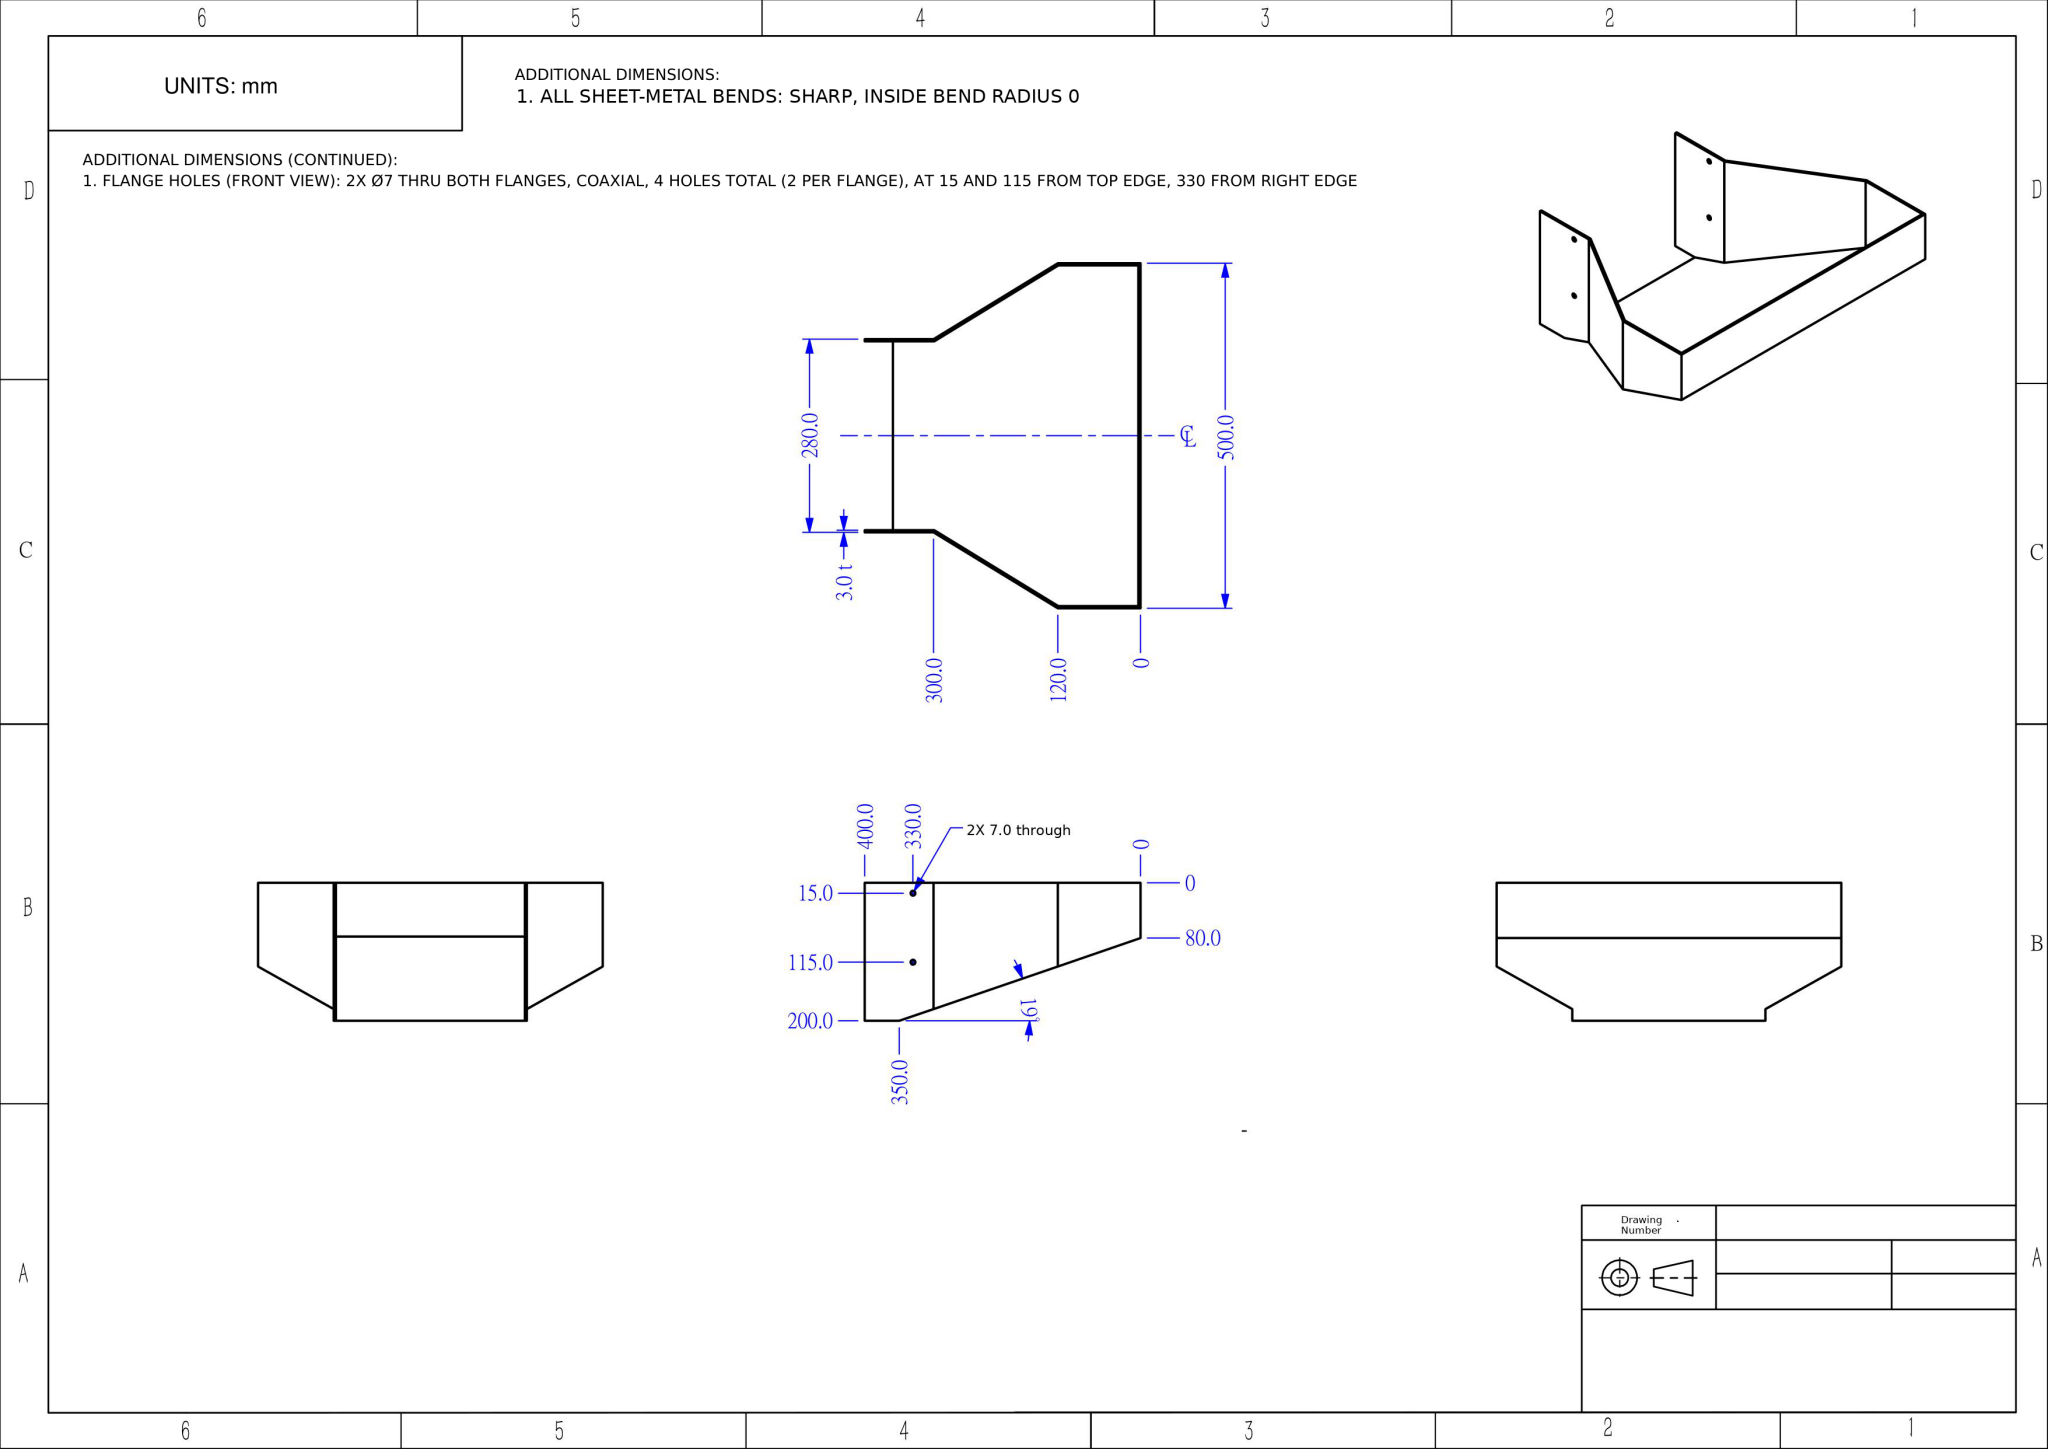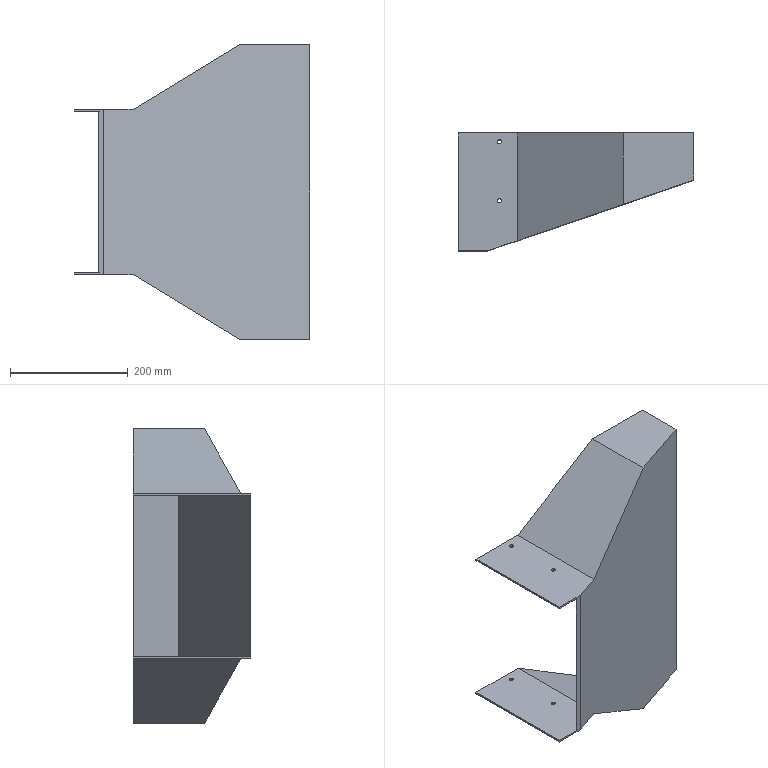Part | NX | mm | 1 solid | 28 faces | box 400 x 200 x 500 mm | volume 950450 mm3 | plane 20 | cylinder 8 | commonest cylinder face diameters 7 x8